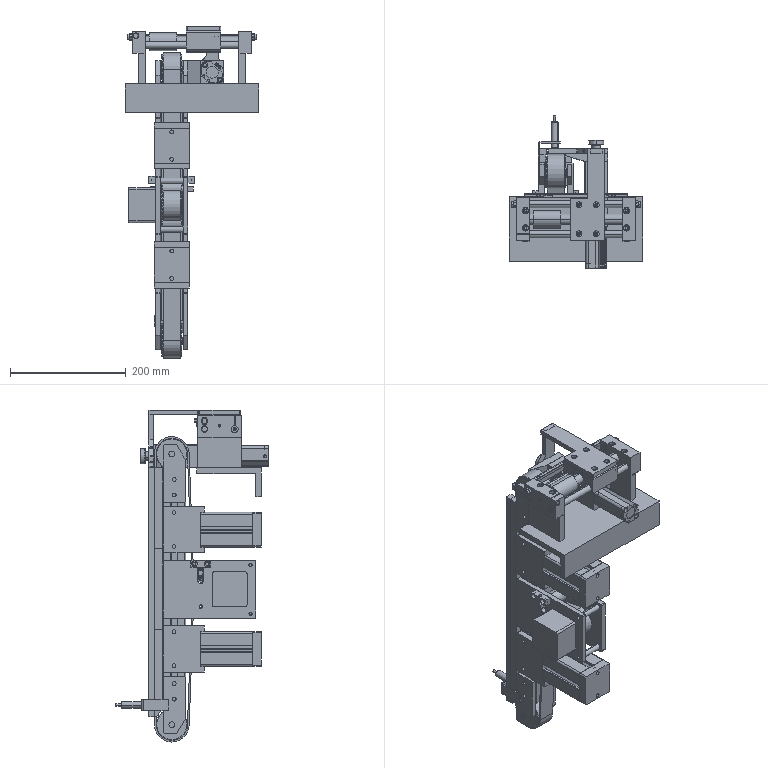Assembly | SolidWorks | mm | 76 component files | 76 solids | 2647 faces | box 230 x 263.7 x 574 mm | volume 3326857 mm3 | plane 1099 | cylinder 1045 | cone 211 | torus 156 | spline 136 | commonest cylinder face diameters 2 x175 10 x104 22.2 x68 13.9 x68 12 x46 6.6 x40 4 x39 26 x34
Bill of materials:
4040-400 | 1 |  | Long straight prismatic extrusion with a square slotted cross-section: one open slot centered on each of the four sides, a round hole near each corner, a central round bore with four radial notches, and diagonal webs linking the core to the corner sections.
60Step | 1 |  | Box-shaped body with a square end face. That face has four small corner holes, a short circular raised boss, and a plain cylindrical shaft sticking out from its center; the body's long edges are rounded.
AOB02-H6060YE-L90 | 2 |  | Short straight prismatic extrusion with a square cross-section and rounded outer corners. There is one undercut T-shaped slot centred on each of the four faces. The core is a central round bore with four small radial notches. Diagonal webs join the core to four hollow corner chambers, and the slot-side pockets have chamfered walls. The cross-section stays the same along the length, and both ends are cut flat.
B6000RS(brandSKF,InnerDiameter10,OuterDiameter26,Thickness8) | 17 | 45 | Short thick annular ring (a cylinder with a central round through bore). One face may have a faint circular groove or step between the bore and the outer diameter.
BAR6800 | 4 |  | Annular ring with a large central bore and stepped concentric recesses on the end face, giving distinct outer-ring, middle-band and inner-ring zones.
BAU6001Z | 2 |  | Annular ring with a central bore and concentric stepped recesses on the end face. Compared with the bore, the ring section is wider than in unnamed part.
CHEN123-AA-21 | 1 |  | Straight angle section with an L-shaped cross-section: two perpendicular flat legs of roughly equal thickness, one leg clearly longer than the other, extruded along a constant length.
CHEN123-AA-23 | 1 |  | Flat plate with an L- or stepped outline: a wider rectangular base with four through holes in a rectangular pattern, and a narrower arm running from one side of the base that ends in an open rectangular notch.
CHEN123-AA-24 | 1 |  | Flat bracket plate with two perpendicular straight arms joined by a diagonal web. A large semicircular cutout sits at the outer side of the joint, and a short angled tab runs beside the cutout. A small hole is drilled into one edge face.
CDQ2B20-40-L-M9B(0_0)_BODY | 1 |  | Prismatic extrusion with a roughly square cross-section and cut-off (chamfered) corners. Two diagonally opposite corners have round through holes. Other corner and edge areas have small circular slots with narrow openings, and parallel longitudinal grooves run along one face.
CDQ2B20-40-M9B(0_0)_CYROD | 1 |  | Headed cylindrical pin: a straight round shank with a larger flat disc head at one end and a flat cut on the side of the shank near the other end.
CHEN123-AA-25 | 1 |  | Rectangular block with a square cross-section and small chamfers on the long edges, with a single round bore running the full length through its center.
D-M9B(CQ2_20) | 2 |  | Elongated prismatic body: a cylinder merged with a square-cornered rectangular section along its full length. A smaller-diameter round pin sticks out of one end, and a slotted screw-head-like feature sits on the flat face near the other end.
CHEN123-AA-26 | 1 |  | Stepped cylindrical pin with three coaxial diameters: a large short disk-like head, a mid-diameter section and a small-diameter tip. All step edges are chamfered.
CHEN123-AA-27 | 1 |  | Stepped cylindrical shaft: a larger-diameter main section steps down to a smaller-diameter section, ending in a short chamfered tip of smaller diameter again. The opposite end has a slot cut across the end face and a circumferential groove near the end.
CHEN123-AA-28 | 1 |  | Small block with one circular through-hole. One end has an angled, tapered face. A rectangular step or notch gives one profile an L shape.
OFG01-d20-L30 | 1 |  | Thin-walled cylindrical sleeve (tube) with a through bore. The outer edges are chamfered, with a larger taper chamfer at one end.
CHEN123-AA-22 | 2 |  | Plain rectangular block or plate with no visible holes or features.
CS1-E | 2 |  | Long rectangular bar with a cylindrical rod sticking out of one end along its axis. The top face has a shallow notch and a rectangular pocket holding a small round raised feature.
RMT-16X100-S(0)_body | 1 |  | Rectangular block. The top face has two shallow lengthwise grooves and four small holes with conical ends. The end face has a large central bore with concentric stepped or counterbored rings, two smaller round through-holes on either side, and small partial holes near the upper corners. The corners are chamfered and the edge profile is notched.
RMT-16X100-S(0)-G-2_rod | 1 |  | Multi-body-looking frame: two rectangular end blocks joined by parallel rods (two slimmer outer rods and one larger central rod). A cylindrical sleeve sits on the central rod, and a rectangular bar runs along one side between the blocks. Hex-shaped protrusions stick out of the outer faces of the end blocks.
Belt | 1 |  | Thin strip of constant thickness bent into a closed elongated loop. Both long ends are rounded, and a small rounded loop sticks out sideways at mid-length. It looks like an extruded wire-like or band profile.
CHEN123-AA-06 | 4 |  | Flat elongated plate. One end has a large angled corner cut and the other corners have small chamfers. It has three circular through-holes: a larger one near the angled end and two smaller ones along the centerline.
CHEN123-AA-07 | 2 |  | U-shaped channel bracket: a base with two parallel upright walls. Each wall has two small through-holes. The wall profile has a rectangular notch or ledge along one edge, and the opposite corners are chamfered.
CHEN123-AA-08 | 2 |  | Thick, nearly square rectangular block/plate with four chamfered corners and two through-holes on the centerline near opposite edges.
CHEN123-AA-09 | 2 |  | Short, thick-walled cylindrical ring/sleeve with a concentric through-bore. Length is slightly greater than outer diameter.
CHEN123-AA-10 | 2 |  | Solid stepped cylindrical shaft: a larger-diameter center section with a smaller-diameter journal at each end.
CHEN123-AA-11 | 1 |  | Thin rectangular plate with slightly rounded corners, one elongated slot, and one small round through-hole.
CHEN123-AA-12 | 1 |  | Thin rectangular plate with rounded corners. It has one large circular through-opening, a square pattern of four small holes around it, two holes near the corners at one end, one elongated slot, and one additional round hole.
CHEN123-AA-13 | 1 |  | Spool- or pulley-like body: a cylindrical center drum with a slightly larger flange at each end and a central keyed bore.
CHEN123-AA-14 | 2 |  | Cylindrical tube/sleeve with a concentric through-bore and chamfered outer edges at both ends. Length is greater than outer diameter.
CHEN123-AA-15 | 2 |  | Long slender tube with a concentric through-bore and small chamfers on the outer edges at both ends.
CHEN123-AA-16 | 1 |  | Rectangular bar/plate with a shallow rectangular step or recess along the middle of one long edge, and an angled bevel along one end edge.
CHEN123-AA-17 | 2 |  | Rectangular bar/plate with a shallow rectangular step or recess along the middle of one long edge. The other edges are square.
CHEN123-AA-18 | 1 |  | Very thin rectangular sheet/strip with one end edge beveled to a sharp, blade-like edge.
CHEN123-AA-19 | 1 |  | Very thin rectangular sheet/strip with one end edge beveled. The bevel is on the side opposite to unnamed part.
CHEN123-AA-20 | 1 |  | L-shaped bent flat plate (angle bracket form) of uniform thin thickness, with a roughly 90-degree bend and a single round through hole near the free end of one leg.
CHEN123-AA-29 | 1 |  | Hollow cylindrical tube or sleeve with chamfered ends, a central through bore, and a short flat or reduced section cut along the outside near one end.
CHEN123-AA-36 | 1 |  | Straight bar with square-section ends and a coaxial cylindrical middle section that is slightly larger than the square end width.
CHEN123-AA-37 | 2 |  | Solid rectangular block with three round through holes: one through the top face at the center, and two parallel holes through the long side face near each end.
ZJG28 | 1 |  | Solid stepped cylindrical pin: a larger cylindrical body with small edge chamfers, and a smaller-diameter coaxial cylindrical spigot sticking out of one end.
Mates:
1. coincident | 4040-400-1 face at (20, 6.101, -400) dir (1, 0, 0) | CHEN123-AA-06-1 face at (20, 0.000896, 0) dir (-1, 0, 0)
2. distance | CHEN123-AA-06-1 face at (28, 19.001, 50) dir (0, 1, 0) | 4040-400-1 face at (18, 20.001, -400) dir (0, 1, 0)
3. distance | CHEN123-AA-06-1 face at (28, -18.999, 50) dir (0, 0, 1) | 4040-400-1 face at (-18, 18.001, 0) dir (0, 0, 1)
4. coincident | 4040-400-1 face at (-20, 18.001, -400) dir (-1, 0, 0) | CHEN123-AA-06-2 face at (-20, 0.000896, 0) dir (1, 0, 0)
5. coincident | CHEN123-AA-06-1 face at (28, 19.001, 50) dir (0, 1, 0) | CHEN123-AA-06-2 face at (-20, 19.001, 50) dir (0, 1, 0)
6. coincident | CHEN123-AA-06-1 face at (28, -18.999, 50) dir (0, 0, 1) | CHEN123-AA-06-2 face at (-20, -18.999, 50) dir (0, 0, 1)
7. coincident | 4040-400-1 face at (20, 6.101, -400) dir (1, 0, 0) | CHEN123-AA-07-1 face at (20, -35.999, -57) dir (-1, 0, 0)
8. coincident | CHEN123-AA-06-1 face at (28, 19.001, 50) dir (0, 1, 0) | CHEN123-AA-07-1 face at (20, 19.001, -57) dir (0, 1, 0)
9. distance | CHEN123-AA-07-1 face at (-0.0005, -51.999, -57) dir (0, 0, 1) | 4040-400-1 face at (-18, 18.001, 0) dir (0, 0, 1)
10. coincident | CHEN123-AA-07-1 face at (30, 19.001, -57) dir (1, 0, 0) | CHEN123-AA-07-2 face at (30, 19.001, -263) dir (1, 0, 0)
11. coincident | CHEN123-AA-07-1 face at (20, 19.001, -57) dir (0, 1, 0) | CHEN123-AA-07-2 face at (20, 19.001, -263) dir (0, 1, 0)
12. distance | CHEN123-AA-07-2 face at (-0.0005, -51.999, -343) dir (0, 0, -1) | 4040-400-1 face at (-18, 18.001, -400) dir (0, 0, -1)
13. coincident | CHEN123-AA-07-1 face at (30, -45.999, -127) dir (0, -1, 0) | AOB02-H6060YE-L90-1 face at (-27, -45.999, -70) dir (0, 1, 0)
14. coincident | CHEN123-AA-07-1 face at (30, 19.001, -57) dir (1, 0, 0) | AOB02-H6060YE-L90-1 face at (30, -135.999, -103.1) dir (1, 0, 0)
15. coincident | CHEN123-AA-07-1 face at (30, -51.999, -127) dir (0, 0, 1) | AOB02-H6060YE-L90-1 face at (-6.101, -135.999, -127) dir (0, 0, -1)
16. coincident | CHEN123-AA-07-2 face at (30, 19.001, -263) dir (1, 0, 0) | AOB02-H6060YE-L90-2 face at (30, -135.999, -309.1) dir (1, 0, 0)
17. coincident | CHEN123-AA-07-2 face at (30, -45.999, -333) dir (0, -1, 0) | AOB02-H6060YE-L90-2 face at (-27, -45.999, -276) dir (0, 1, 0)
18. coincident | CHEN123-AA-07-2 face at (30, -51.999, -333) dir (0, 0, 1) | AOB02-H6060YE-L90-2 face at (27, -135.999, -333) dir (0, 0, -1)
19. coincident | AOB02-H6060YE-L90-1 face at (-27, -135.999, -70) dir (0, -1, 0) | CHEN123-AA-08-1 face at (-0.0005, -135.999, -97) dir (0, 1, 0)
20. coincident | AOB02-H6060YE-L90-1 face at (30, -135.999, -70) dir (1, 0, 0) | CHEN123-AA-08-1 face at (30, -135.999, -67) dir (1, 0, 0)
21. coincident | AOB02-H6060YE-L90-1 face at (6.099, -135.999, -67) dir (0, 0, 1) | CHEN123-AA-08-1 face at (-30, -135.999, -67) dir (0, 0, 1)
22. coincident | AOB02-H6060YE-L90-2 face at (30, -135.999, -276) dir (1, 0, 0) | CHEN123-AA-08-2 face at (30, -135.999, -273) dir (1, 0, 0)
23. coincident | AOB02-H6060YE-L90-2 face at (6.099, -135.999, -273) dir (0, 0, 1) | CHEN123-AA-08-2 face at (-30, -135.999, -273) dir (0, 0, 1)
24. coincident | AOB02-H6060YE-L90-2 face at (-27, -135.999, -276) dir (0, -1, 0) | CHEN123-AA-08-2 face at (-0.0005, -135.999, -303) dir (0, 1, 0)
25. concentric | CHEN123-AA-06-1 face at (20, 4.001, 34) dir (1, 0, 0) r 5 | CHEN123-AA-09-1 face at (17.5, 4.001, 34) dir (-1, 0, 0) r 27
26. distance | CHEN123-AA-09-1 face at (17.5, 4.001, 34) dir (1, 0, 0) | CHEN123-AA-06-1 face at (20, 0.000896, 0) dir (-1, 0, 0)
27. concentric | CHEN123-AA-06-3 face at (28, 4.001, -434) dir (-1, 0, 0) r 5 | CHEN123-AA-09-2 face at (17.5, 4.001, -434) dir (-1, 0, 0) r 27
28. coincident | CHEN123-AA-09-1 face at (17.5, 4.001, 34) dir (1, 0, 0) | CHEN123-AA-09-2 face at (17.5, 4.001, -434) dir (1, 0, 0)
29. concentric | CHEN123-AA-06-1 face at (20, 4.001, 34) dir (1, 0, 0) r 5 | CHEN123-AA-10-1 face at (18, 4.001, 34) dir (-1, 0, 0) r 6
30. coincident | CHEN123-AA-06-1 face at (28, 0.000896, 0) dir (1, 0, 0) | CHEN123-AA-10-1 face at (28, 4.001, 34) dir (1, 0, 0)
31. concentric | CHEN123-AA-06-3 face at (28, 4.001, -434) dir (-1, 0, 0) r 5 | CHEN123-AA-10-2 face at (18, 4.001, -434) dir (-1, 0, 0) r 6
32. coincident | CHEN123-AA-06-3 face at (28, 0.000896, -400) dir (1, 0, 0) | CHEN123-AA-10-2 face at (28, 4.001, -434) dir (1, 0, 0)
33. concentric | CHEN123-AA-09-1 face at (17.5, 4.001, 34) dir (-1, 0, 0) r 27 | BAU6001Z-1 face at (-7.801, 4.001, 34) dir (-1, 0, 0) r 14
34. coincident | CHEN123-AA-09-1 face at (-7.5, 4.001, 34) dir (-1, 0, 0) | BAU6001Z-1 face at (-7.5, 15.392, 31.117) dir (1, 0, 0)
35. concentric | CHEN123-AA-09-1 face at (17.5, 4.001, 34) dir (-1, 0, 0) r 27 | BAU6001Z-2 face at (15.2, 4.001, 34) dir (-1, 0, 0) r 14
36. coincident | CHEN123-AA-09-1 face at (7.5, 4.001, 34) dir (1, 0, 0) | BAU6001Z-2 face at (7.5, 15.946, 40.708) dir (-1, 0, 0)
37. coincident | 4040-400-1 face at (20, 6.101, -400) dir (1, 0, 0) | CHEN123-AA-11-1 face at (20, -60.999, -200) dir (-1, 0, 0)
38. coincident | CHEN123-AA-07-1 face at (20, 19.001, -57) dir (0, 1, 0) | CHEN123-AA-11-1 face at (20, 19.001, -250) dir (0, 1, 0)
39. distance | CHEN123-AA-11-1 face at (20, -140.999, -150) dir (0, 0, 1) | 4040-400-1 face at (-18, 18.001, 0) dir (0, 0, 1)
40. coincident | 4040-400-1 face at (-20, 18.001, -400) dir (-1, 0, 0) | CHEN123-AA-12-1 face at (-20, -60.999, -200) dir (1, 0, 0)
41. coincident | CHEN123-AA-11-1 face at (20, 19.001, -250) dir (0, 1, 0) | CHEN123-AA-12-1 face at (-20, 19.001, -150) dir (0, 1, 0)
42. coincident | CHEN123-AA-11-1 face at (20, -140.999, -150) dir (0, 0, 1) | CHEN123-AA-12-1 face at (-20, -140.999, -150) dir (0, 0, 1)
43. concentric | CHEN123-AA-12-1 face at (-8.001, -95.999, -200) dir (-1, 0, 0) r 19 | 60Step-1 face at (-6.401, -95.999, -200) dir (-1, 0, 0) r 4
44. coincident | CHEN123-AA-12-1 face at (-28, -60.999, -200) dir (-1, 0, 0) | 60Step-1 face at (-28, -95.999, -200) dir (1, 0, 0)
45. parallel | CHEN123-AA-12-1 face at (-20, -140.999, -150) dir (0, 0, 1) | 60Step-1 face at (-28, -65.999, -170) dir (0, 0, 1)
46. concentric | 60Step-1 face at (-6.401, -95.999, -200) dir (-1, 0, 0) r 4 | CHEN123-AA-13-1 face at (-16, -95.999, -200) dir (1, 0, 0) r 20
47. width | CHEN123-AA-12-1 face at (-28, -60.999, -200) dir (-1, 0, 0) | CHEN123-AA-11-1 face at (28, -60.999, -200) dir (1, 0, 0) | CHEN123-AA-13-1 face at (18, -95.999, -200) dir (1, 0, 0) | CHEN123-AA-13-1 face at (-18, -95.999, -200) dir (-1, 0, 0)
48. concentric | CHEN123-AA-12-1 face at (-20, -45.999, -230) dir (-1, 0, 0) r 3 | CHEN123-AA-14-1 face at (-17.5, -45.999, -230) dir (1, 0, 0) r 12.5
49. distance | CHEN123-AA-14-1 face at (-17.5, -45.999, -230) dir (-1, 0, 0) | CHEN123-AA-12-1 face at (-20, -60.999, -200) dir (1, 0, 0)
50. symmetric | CHEN123-AA-12-1 face at (-20, -50.999, -160) dir (0, 1, 0) | CHEN123-AA-12-1 face at (-20, -40.999, -160) dir (0, -1, 0) | CHEN123-AA-14-2 plane at (-0.0005, -45.999, -172) dir (0, 1, 0)
51. coincident | CHEN123-AA-14-1 face at (17.5, -45.999, -230) dir (1, 0, 0) | CHEN123-AA-14-2 face at (17.5, -45.999, -172) dir (1, 0, 0)
52. distance | CHEN123-AA-14-2 plane at (-0.0005, -45.999, -172) dir (0, 0, 1) | CHEN123-AA-12-1 face at (-20, -140.999, -150) dir (0, 0, 1)
53. concentric | CHEN123-AA-14-2 face at (12.3, -45.999, -172) dir (1, 0, 0) r 9.5 | BAR6800-1 face at (17.2, -45.999, -172) dir (-1, 0, 0) r 9.5
54. coincident | CHEN123-AA-14-2 face at (17.5, -45.999, -172) dir (1, 0, 0) | BAR6800-1 face at (17.5, -37.815, -172) dir (1, 0, 0)
55. concentric | CHEN123-AA-14-2 face at (-12.3, -45.999, -172) dir (-1, 0, 0) r 9.5 | BAR6800-2 face at (-12.8, -45.999, -172) dir (-1, 0, 0) r 9.5
56. coincident | CHEN123-AA-14-2 face at (-17.5, -45.999, -172) dir (-1, 0, 0) | BAR6800-2 face at (-17.5, -36.799, -172) dir (-1, 0, 0)
57. concentric | CHEN123-AA-14-1 face at (-17.5, -45.999, -230) dir (1, 0, 0) r 12.5 | BAR6800-3 face at (-12.8, -45.999, -230) dir (-1, 0, 0) r 9.5
58. coincident | CHEN123-AA-14-1 face at (-17.5, -45.999, -230) dir (-1, 0, 0) | BAR6800-3 face at (-17.5, -46.262, -239.196) dir (-1, 0, 0)
59. concentric | CHEN123-AA-14-1 face at (12.3, -45.999, -230) dir (1, 0, 0) r 9.5 | BAR6800-4 face at (17.2, -45.999, -230) dir (-1, 0, 0) r 9.5
60. coincident | CHEN123-AA-14-1 face at (17.5, -45.999, -230) dir (1, 0, 0) | BAR6800-4 face at (17.5, -37.815, -230) dir (1, 0, 0)
61. concentric | CHEN123-AA-09-2 face at (17.5, 4.001, -434) dir (-1, 0, 0) r 27 | Belt-1 sketch segment at (-0.0005, 4.001, -434) dir (-1, 0, 0) r 27
62. parallel | 4040-400-1 face at (18, 20.001, -400) dir (0, 1, 0) | Belt-1 plane at (-0.0005, 4.001, -329.44) dir (0, 1, 0)
63. symmetric | CHEN123-AA-09-2 face at (-17.5, 4.001, -434) dir (-1, 0, 0) | CHEN123-AA-09-2 face at (17.5, 4.001, -434) dir (1, 0, 0) | Belt-1 plane at (-0.0005, 4.001, -329.44) dir (-1, 0, 0)
64. concentric | CHEN123-AA-12-1 face at (-28, -132.097, -242.036) dir (-1, 0, 0) r 2.75 | CHEN123-AA-15-1 face at (-20, -132.097, -242.036) dir (1, 0, 0) r 5
65. coincident | CHEN123-AA-12-1 face at (-20, -60.999, -200) dir (1, 0, 0) | CHEN123-AA-15-1 face at (-20, -132.097, -242.036) dir (-1, 0, 0)
66. concentric | CHEN123-AA-12-1 face at (-28, -132.097, -158.067) dir (-1, 0, 0) r 2.75 | CHEN123-AA-15-2 face at (-20, -132.097, -158.067) dir (1, 0, 0) r 5
67. coincident | CHEN123-AA-11-1 face at (20, -60.999, -200) dir (-1, 0, 0) | CHEN123-AA-15-2 face at (20, -132.097, -158.067) dir (1, 0, 0)
68. distance | 4040-400-1 face at (-20, 18.001, -400) dir (-1, 0, 0) | CHEN123-AA-16-1 face at (-28, 20.001, -420) dir (-1, 0, 0)
69. coincident | 4040-400-1 face at (-6.101, 20.001, -400) dir (0, 1, 0) | CHEN123-AA-16-1 face at (-0.0005, 20.001, -345) dir (0, -1, 0)
70. distance | CHEN123-AA-16-1 face at (28, 20.001, -420) dir (0, 0, -1) | 4040-400-1 face at (-18, 18.001, -400) dir (0, 0, -1)
71. coincident | 4040-400-1 face at (-6.101, 20.001, -400) dir (0, 1, 0) | CHEN123-AA-17-1 face at (-0.0005, 20.001, -200) dir (0, -1, 0)
72. coincident | CHEN123-AA-16-1 face at (-28, 20.001, -420) dir (-1, 0, 0) | CHEN123-AA-17-1 face at (-28, 20.001, -270) dir (-1, 0, 0)
73. coincident | CHEN123-AA-16-1 face at (28, 20.001, -270) dir (0, 0, 1) | CHEN123-AA-17-1 face at (28, 20.001, -270) dir (0, 0, -1)
74. coincident | CHEN123-AA-17-1 face at (-28, 20.001, -270) dir (-1, 0, 0) | CHEN123-AA-17-2 face at (-28, 20.001, -130) dir (-1, 0, 0)
75. coincident | 4040-400-1 face at (-6.101, 20.001, -400) dir (0, 1, 0) | CHEN123-AA-17-2 face at (-0.0005, 20.001, -60) dir (0, -1, 0)
76. coincident | CHEN123-AA-17-1 face at (28, 20.001, -130) dir (0, 0, 1) | CHEN123-AA-17-2 face at (28, 20.001, -130) dir (0, 0, -1)
77. coincident | CHEN123-AA-16-1 face at (-0.0005, 34.001, -345) dir (0, 1, 0) | CHEN123-AA-18-1 face at (-22.25, 34.001, -205) dir (0, -1, 0)
78. coincident | CHEN123-AA-16-1 face at (-28, 20.001, -420) dir (-1, 0, 0) | CHEN123-AA-18-1 face at (-28, 44.001, -420) dir (-1, 0, 0)
79. coincident | CHEN123-AA-17-2 face at (28, 20.001, 10) dir (0, 0, 1) | CHEN123-AA-18-1 face at (-28, 44.001, 10) dir (0, 0, 1)
80. coincident | CHEN123-AA-16-1 face at (-0.0005, 34.001, -345) dir (0, 1, 0) | CHEN123-AA-19-1 face at (22.25, 34.001, -205) dir (0, -1, 0)
81. coincident | CHEN123-AA-16-1 face at (28, 20.001, -420) dir (1, 0, 0) | CHEN123-AA-19-1 face at (28, 44.001, -420) dir (1, 0, 0)
82. coincident | CHEN123-AA-16-1 face at (28, 20.001, -420) dir (0, 0, -1) | CHEN123-AA-19-1 face at (16.5, 44.001, -420) dir (0, 0, -1)
83. coincident | Belt-1 face at (-15.001, 34.001, -434) dir (0, 1, 0) | B6000RS(brandSKF,InnerDiameter10,OuterDiameter26,Thickness8)-1 face at (-6.125, 34.001, -405) dir (0, -1, 0)
84. symmetric | CHEN123-AA-18-1 face at (-28, 44.001, -420) dir (-1, 0, 0) | CHEN123-AA-19-1 face at (28, 44.001, -420) dir (1, 0, 0) | B6000RS(brandSKF,InnerDiameter10,OuterDiameter26,Thickness8)-1 plane at (-0.0005, 34.001, -405) dir (-1, 0, 0)
85. distance | B6000RS(brandSKF,InnerDiameter10,OuterDiameter26,Thickness8)-1 plane at (-0.0005, 34.001, -405) dir (0, 0, 1) | CHEN123-AA-18-1 face at (-28, 44.001, -420) dir (0, 0, -1)
86. coincident | CHEN123-AA-06-4 face at (-28, 0.000896, -400) dir (-1, 0, 0) | CHEN123-AA-20-1 face at (-28, 9.001, -410) dir (1, 0, 0)
87. distance | CHEN123-AA-20-1 face at (-27.264, 53.264, -410) dir (0, 0, -1) | CHEN123-AA-06-4 face at (-28, -18.999, -450) dir (0, 0, -1)
88. distance | CHEN123-AA-20-1 face at (-30, 9.001, -410) dir (0, -1, 0) | CHEN123-AA-06-4 face at (-28, 19.001, -450) dir (0, 1, 0)
89. concentric | CHEN123-AA-20-1 face at (-2.001, 56.001, -400) dir (0, 1, 0) r 6 | ZJG28-1 face at (-2.001, 91.001, -400) dir (0, -1, 0) r 6
90. distance | ZJG28-1 face at (-2.001, 46.001, -400) dir (0, -1, 0) | CHEN123-AA-20-1 face at (-28, 54.001, -410) dir (0, -1, 0)
91. coincident | CHEN123-AA-08-1 face at (-0.0005, -150.999, -97) dir (0, -1, 0) | BearingLiftingModule-1/CHEN123-AA-21-1 face at (-80.001, -150.999, 10) dir (0, -1, 0)
92. distance | BearingLiftingModule-1/CHEN123-AA-21-1 face at (-80.001, -150.999, -40) dir (0, 0, -1) | CHEN123-AA-08-1 face at (-30, -135.999, -67) dir (0, 0, 1)
93. distance | BearingLiftingModule-1/CHEN123-AA-21-1 face at (-80.001, -150.999, 10) dir (-1, 0, 0) | CHEN123-AA-08-1 face at (-30, -135.999, -67) dir (-1, 0, 0)
94. concentric | CHEN123-AA-14-1 face at (17.5, -45.999, -230) dir (-1, 0, 0) r 6 | CHEN123-AA-29-1 face at (-20, -45.999, -230) dir (1, 0, 0) r 5
95. coincident | CHEN123-AA-11-1 face at (20, -60.999, -200) dir (-1, 0, 0) | CHEN123-AA-29-1 face at (20, -45.999, -230) dir (1, 0, 0)
96. concentric | BAR6800-2 face at (-12.8, -45.999, -172) dir (-1, 0, 0) r 5 | CHEN123-AA-36-1 face at (-37.501, -45.999, -172) dir (1, 0, 0) r 5
97. coincident | CHEN123-AA-12-1 face at (-28, -60.999, -200) dir (-1, 0, 0) | CHEN123-AA-37-1 face at (-28, -45.999, -156) dir (1, 0, 0)
98. coincident | CHEN123-AA-12-1 face at (-20, -140.999, -150) dir (0, 0, 1) | CHEN123-AA-37-1 face at (-40.001, -62.999, -150) dir (0, 0, 1)
99. width | CHEN123-AA-37-1 face at (-40.001, -28.999, -162) dir (0, 1, 0) | CHEN123-AA-37-1 face at (-40.001, -62.999, -162) dir (0, -1, 0) | CHEN123-AA-12-1 face at (-20, -40.999, -160) dir (0, -1, 0) | CHEN123-AA-12-1 face at (-20, -50.999, -160) dir (0, 1, 0)
100. coincident | CHEN123-AA-11-1 face at (28, -60.999, -200) dir (1, 0, 0) | CHEN123-AA-37-2 face at (28, -45.999, -156) dir (-1, 0, 0)
101. coincident | CHEN123-AA-11-1 face at (20, -140.999, -150) dir (0, 0, 1) | CHEN123-AA-37-2 face at (39.999, -62.999, -150) dir (0, 0, 1)
102. coincident | CHEN123-AA-37-1 face at (-40.001, -28.999, -162) dir (0, 1, 0) | CHEN123-AA-37-2 face at (39.999, -28.999, -150) dir (0, 1, 0)
103. width | CHEN123-AA-36-1 face at (37.499, -45.999, -172) dir (1, 0, 0) | CHEN123-AA-36-1 face at (-37.501, -45.999, -172) dir (-1, 0, 0) | CHEN123-AA-12-1 face at (-28, -60.999, -200) dir (-1, 0, 0) | CHEN123-AA-11-1 face at (28, -60.999, -200) dir (1, 0, 0)
104. concentric | BearingLiftingModule-1/CylinderLiftingModule-1/CHEN123-AA-27-1 face at (69.999, 56.301, 30) dir (0, -1, 0) r 5 | B6000RS(brandSKF,InnerDiameter10,OuterDiameter26,Thickness8)-17 face at (69.999, 54.301, 30) dir (0, 1, 0) r 5
105. coincident | BearingLiftingModule-1/CylinderLiftingModule-1/CHEN123-AA-27-1 face at (69.999, 50.301, 30) dir (0, 1, 0) | B6000RS(brandSKF,InnerDiameter10,OuterDiameter26,Thickness8)-17 face at (63.874, 50.301, 30) dir (0, -1, 0)
106. coincident | CHEN123-AA-21-1 face at (0, 0, 115) dir (1, 0, 0) | RMT16X100S_0_+_CS1-G-2-1/CHEN123-AA-22-2 face at (0, 72.5, -87) dir (-1, 0, 0)
107. width | CHEN123-AA-21-1 face at (0, 0, 115) dir (0, 0, 1) | CHEN123-AA-21-1 face at (0, 0, -115) dir (0, 0, -1) | RMT16X100S_0_+_CS1-G-2-1/RMT-16X100-S(0)-G-2_rod-1 face at (73, 72.5, -103.5) dir (0, 0, -1) | RMT16X100S_0_+_CS1-G-2-1/RMT-16X100-S(0)-G-2_rod-1 face at (71.5, 72.5, 103.5) dir (0, 0, 1)
108. distance | RMT16X100S_0_+_CS1-G-2-1/CHEN123-AA-22-2 face at (52, 110, -81) dir (0, 1, 0) | CHEN123-AA-21-1 face at (-10, 112, 115) dir (0, 1, 0)
109. coincident | RMT16X100S_0_+_CS1-G-2-1/RMT-16X100-S(0)_body-1 face at (92, 105.672, -50) dir (1, 0, 0) | CHEN123-AA-23-1 face at (92, 115.5, -20) dir (-1, 0, 0)
110. coincident | RMT16X100S_0_+_CS1-G-2-1/RMT-16X100-S(0)_body-1 face at (71.5, 72.5, -50) dir (0, 0, -1) | CHEN123-AA-23-1 face at (100, 36.5, -50) dir (0, 0, -1)
111. coincident | RMT16X100S_0_+_CS1-G-2-1/RMT-16X100-S(0)_body-1 face at (89.172, 36.5, -50) dir (0, -1, 0) | CHEN123-AA-23-1 face at (100, 36.5, 10) dir (0, -1, 0)
112. coincident | CHEN123-AA-23-1 face at (90, 186.5, -25) dir (0, 1, 0) | CHEN123-AA-24-1 face at (54.5, 186.5, -0.5) dir (0, -1, 0)
113. coincident | CHEN123-AA-23-1 face at (90, 186.5, -45) dir (0, 0, 1) | CHEN123-AA-24-1 face at (100, 186.5, -45) dir (0, 0, -1)
114. coincident | CHEN123-AA-23-1 face at (100, 115.5, -20) dir (1, 0, 0) | CHEN123-AA-24-1 face at (100, 194.5, 49) dir (1, 0, 0)
115. coincident | CHEN123-AA-21-1 face at (0, 0, 115) dir (1, 0, 0) | CylinderLiftingModule-1/CDQ2B20-40DZ-L-M9B_0_0_0-1/CHEN123-AA-25-1 face at (0, 59.8, -55) dir (-1, 0, 0)
116. distance | CHEN123-AA-24-1 face at (54.5, 194.5, -0.5) dir (0, 1, 0) | CylinderLiftingModule-1/CHEN123-AA-28-1 face at (20, 186.3, -18.5) dir (0, 1, 0)
117. distance | CylinderLiftingModule-1/CDQ2B20-40DZ-L-M9B_0_0_0-1/CHEN123-AA-25-1 face at (0, 59.8, -55) dir (0, 0, -1) | CHEN123-AA-21-1 face at (0, 0, -115) dir (0, 0, -1)
118. concentric | CDQ2B20-40DZ-L-M9B_0_0_0-1/CHEN123-AA-25-1 face at (-50, 0, 0) dir (-1, 0, 0) r 14 | OFG01-d20-L30-1 face at (-50, 0, 0) dir (-1, 0, 0) r 14
119. coincident | CDQ2B20-40DZ-L-M9B_0_0_0-1/CHEN123-AA-25-1 face at (-80, 0, 0) dir (-1, 0, 0) | OFG01-d20-L30-1 face at (-80, 13.5, 0) dir (-1, 0, 0)
120. concentric | CDQ2B20-40DZ-L-M9B_0_0_0-1/CDQ2B20-40-M9B(0_0)_CYROD-1 face at (30.367, 0, 0) dir (-1, 0, 0) r 5 | CHEN123-AA-26-1 face at (-23.133, 0, 0) dir (-1, 0, 0) r 2.067
121. coincident | CDQ2B20-40DZ-L-M9B_0_0_0-1/CDQ2B20-40-M9B(0_0)_CYROD-1 face at (-29.133, 1.58, -1.937) dir (-1, 0, 0) | CHEN123-AA-26-1 face at (-29.133, 0, 0) dir (1, 0, 0)
122. concentric | CHEN123-AA-26-1 face at (-29.133, 0, 0) dir (-1, 0, 0) r 4 | CHEN123-AA-27-1 face at (-96.133, 0, 0) dir (1, 0, 0) r 10
123. coincident | CHEN123-AA-26-1 face at (-35.133, 0, 0) dir (1, 0, 0) | CHEN123-AA-27-1 face at (-35.133, 11.723, 2.475) dir (-1, 0, 0)
124. coincident | CDQ2B20-40DZ-L-M9B_0_0_0-1/CHEN123-AA-25-1 face at (-113, 0, 0) dir (-1, 0, 0) | CHEN123-AA-28-1 face at (-113, 16.5, 0) dir (1, 0, 0)
125. concentric | CDQ2B20-40DZ-L-M9B_0_0_0-1/CHEN123-AA-25-1 face at (-80, 0, 0) dir (-1, 0, 0) r 15 | CHEN123-AA-28-1 face at (-113, 0, 0) dir (-1, 0, 0) r 8
126. coincident | CDQ2B20-40DZ-L-M9B_0_0_0-1/CHEN123-AA-25-1 face at (0, -20, -20) dir (0, 0, -1) | CHEN123-AA-28-1 face at (-135, 53, -20) dir (0, 0, -1)
127. concentric | CDQ2B20-40-L-M9B(0_0)_BODY-1 face at (55, 0, 0) dir (-1, 0, 0) r 5 | CDQ2B20-40-M9B(0_0)_CYROD-1 face at (54, 0, 0) dir (-1, 0, 0) r 5
128. distance | CDQ2B20-40-M9B(0_0)_CYROD-1 face at (54, 7.902, -6.129) dir (1, 0, 0) | CDQ2B20-40-L-M9B(0_0)_BODY-1 face at (55, 10, 0) dir (-1, 0, 0)
129. coincident | CDQ2B20-40-L-M9B(0_0)_BODY-1 face at (0, -13.081, 13.081) dir (-1, 0, 0) | CHEN123-AA-25-1 face at (0, 0, 0) dir (1, 0, 0)
130. concentric | CDQ2B20-40-M9B(0_0)_CYROD-1 face at (54, 0, 0) dir (-1, 0, 0) r 5 | CHEN123-AA-25-1 face at (-113, 0, 0) dir (1, 0, 0) r 11.5
131. parallel | CDQ2B20-40-L-M9B(0_0)_BODY-1 face at (71.5, 6.466, 18) dir (0, 0, 1) | CHEN123-AA-25-1 face at (0, -20, 20) dir (0, 0, 1)
132. concentric | RMT-16X100-S(0)-G-2_rod-1 face at (207, 26, -4.5) dir (1, 0, 0) r 6 | RMT-16X100-S(0)_body-1 face at (83.5, 26, -4.5) dir (-1, 0, 0) r 6
133. concentric | RMT-16X100-S(0)-G-2_rod-1 face at (207, -26, -4.5) dir (1, 0, 0) r 6 | RMT-16X100-S(0)_body-1 face at (83.5, -26, -4.5) dir (-1, 0, 0) r 6
134. distance | RMT-16X100-S(0)_body-1 face at (23.5, 0, 0) dir (-1, 0, 0) | RMT-16X100-S(0)-G-2_rod-1 face at (22.5, 0, 0) dir (1, 0, 0)
135. coincident | RMT-16X100-S(0)-G-2_rod-1 face at (22.5, -37.5, -19.5) dir (0, 0, -1) | CHEN123-AA-22-1 face at (16.5, 0, -19.5) dir (0, 0, 1)
136. coincident | RMT-16X100-S(0)-G-2_rod-1 face at (22.5, -37.5, 19.5) dir (0, -1, 0) | CHEN123-AA-22-1 face at (10.5, -37.5, -19.5) dir (0, -1, 0)
137. coincident | RMT-16X100-S(0)-G-2_rod-1 face at (22.5, 0, 0) dir (1, 0, 0) | CHEN123-AA-22-1 face at (22.5, -37.5, -19.5) dir (1, 0, 0)
138. coincident | RMT-16X100-S(0)-G-2_rod-1 face at (184.5, 0, 0) dir (-1, 0, 0) | CHEN123-AA-22-2 face at (184.5, -37.5, -19.5) dir (-1, 0, 0)
139. coincident | RMT-16X100-S(0)-G-2_rod-1 face at (184.5, -37.5, 19.5) dir (0, -1, 0) | CHEN123-AA-22-2 face at (184.5, -37.5, -19.5) dir (0, -1, 0)
140. coincident | CHEN123-AA-22-1 face at (16.5, 0, -71.5) dir (0, 0, -1) | CHEN123-AA-22-2 face at (190.5, 0, -71.5) dir (0, 0, -1)